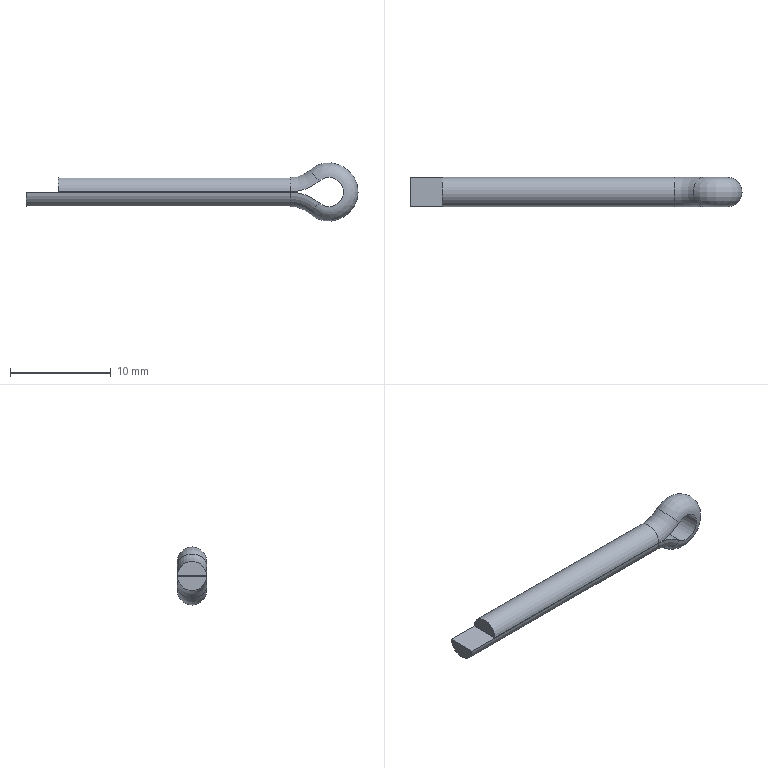Component | NX | COTTER_PIN_2_9X25_2 | 1 solid | 12 faces | box 33 x 2.9 x 5.72 mm | volume 211 mm3 | cylinder 5 | plane 4 | torus 2 | spline 1 | commonest cylinder face diameters 2.9 x2 8.69 x2 2.91 x1
STEP:
#1=VALUE_REPRESENTATION_ITEM('',COUNT_MEASURE(0.));
#2=(LENGTH_UNIT()NAMED_UNIT(*)SI_UNIT(.MILLI.,.METRE.));
#3=UNCERTAINTY_MEASURE_WITH_UNIT(LENGTH_MEASURE(0.0254),#2,'','');
#4=(NAMED_UNIT(*)PLANE_ANGLE_UNIT()SI_UNIT($,.RADIAN.));
#5=PLANE_ANGLE_MEASURE_WITH_UNIT(PLANE_ANGLE_MEASURE(0.01745),#4);
#6=DIMENSIONAL_EXPONENTS(0.,0.,0.,0.,0.,0.,0.);
#7=(CONVERSION_BASED_UNIT('',#5)NAMED_UNIT(#6)PLANE_ANGLE_UNIT());
#8=(NAMED_UNIT(*)SI_UNIT($,.STERADIAN.)SOLID_ANGLE_UNIT());
#9=(GEOMETRIC_REPRESENTATION_CONTEXT(3)GLOBAL_UNCERTAINTY_ASSIGNED_CONTEXT((#3))GLOBAL_UNIT_ASSIGNED_CONTEXT((#2,#7,#8))REPRESENTATION_CONTEXT('',''));
#10=REPRESENTATION('',(#1),#9);
#11=VALUE_REPRESENTATION_ITEM('',COUNT_MEASURE(0.));
#12=REPRESENTATION('',(#11),#9);
#13=CARTESIAN_POINT('',(0.,0.,0.));
#14=DIRECTION('',(0.,0.,1.));
#15=DIRECTION('',(1.,0.,0.));
#16=AXIS2_PLACEMENT_3D('',#13,#14,#15);
#17=SHAPE_REPRESENTATION('',(#16),#9);
#18=CARTESIAN_POINT('',(10.982,22.05,135.805));
#19=VERTEX_POINT('',#18);
#20=CARTESIAN_POINT('',(10.982,24.95,135.805));
#21=VERTEX_POINT('',#20);
#22=CARTESIAN_POINT('',(10.982,22.05,135.805));
#23=DIRECTION('',(0.,1.,0.));
#24=VECTOR('',#23,1.);
#25=LINE('',#22,#24);
#26=EDGE_CURVE('',#19,#21,#25,.T.);
#27=ORIENTED_EDGE('',*,*,#26,.T.);
#28=CARTESIAN_POINT('',(-15.3,24.95,135.805));
#29=VERTEX_POINT('',#28);
#30=CARTESIAN_POINT('',(10.982,24.95,135.805));
#31=DIRECTION('',(-1.,0.,0.));
#32=VECTOR('',#31,1.);
#33=LINE('',#30,#32);
#34=EDGE_CURVE('',#21,#29,#33,.T.);
#35=ORIENTED_EDGE('',*,*,#34,.T.);
#36=CARTESIAN_POINT('',(-15.3,22.05,135.805));
#37=VERTEX_POINT('',#36);
#38=CARTESIAN_POINT('',(-15.3,22.05,135.805));
#39=DIRECTION('',(0.,1.,0.));
#40=VECTOR('',#39,1.);
#41=LINE('',#38,#40);
#42=EDGE_CURVE('',#37,#29,#41,.T.);
#43=ORIENTED_EDGE('',*,*,#42,.F.);
#44=CARTESIAN_POINT('',(10.982,22.05,135.805));
#45=DIRECTION('',(-1.,0.,0.));
#46=VECTOR('',#45,1.);
#47=LINE('',#44,#46);
#48=EDGE_CURVE('',#19,#37,#47,.T.);
#49=ORIENTED_EDGE('',*,*,#48,.F.);
#50=EDGE_LOOP('',(#27,#35,#43,#49));
#51=FACE_OUTER_BOUND('',#50,.T.);
#52=CARTESIAN_POINT('',(10.982,22.05,135.805));
#53=DIRECTION('',(0.,0.,1.));
#54=DIRECTION('',(1.,0.,0.));
#55=AXIS2_PLACEMENT_3D('',#52,#53,#54);
#56=PLANE('',#55);
#57=ADVANCED_FACE('',(#51),#56,.T.);
#58=CARTESIAN_POINT('',(10.982,23.5,135.81));
#59=DIRECTION('',(-1.,0.,-0.));
#60=DIRECTION('',(0.,1.,0.));
#61=AXIS2_PLACEMENT_3D('',#58,#59,#60);
#62=CIRCLE('',#61,1.45);
#63=EDGE_CURVE('',#21,#19,#62,.T.);
#64=ORIENTED_EDGE('',*,*,#63,.T.);
#65=ORIENTED_EDGE('',*,*,#48,.T.);
#66=CARTESIAN_POINT('',(-15.3,23.5,135.81));
#67=DIRECTION('',(-1.,0.,-0.));
#68=DIRECTION('',(0.,1.,0.));
#69=AXIS2_PLACEMENT_3D('',#66,#67,#68);
#70=CIRCLE('',#69,1.45);
#71=EDGE_CURVE('',#29,#37,#70,.T.);
#72=ORIENTED_EDGE('',*,*,#71,.F.);
#73=ORIENTED_EDGE('',*,*,#34,.F.);
#74=EDGE_LOOP('',(#64,#65,#72,#73));
#75=FACE_OUTER_BOUND('',#74,.T.);
#76=CARTESIAN_POINT('',(10.982,23.5,135.81));
#77=DIRECTION('',(-1.,0.,0.));
#78=DIRECTION('',(0.,-1.,0.));
#79=AXIS2_PLACEMENT_3D('',#76,#77,#78);
#80=CYLINDRICAL_SURFACE('',#79,1.45);
#81=ADVANCED_FACE('',(#75),#80,.T.);
#82=CARTESIAN_POINT('',(13.856,22.05,134.719));
#83=VERTEX_POINT('',#82);
#84=CARTESIAN_POINT('',(13.856,24.95,134.719));
#85=VERTEX_POINT('',#84);
#86=CARTESIAN_POINT('',(13.856,22.05,134.719));
#87=DIRECTION('',(0.,1.,0.));
#88=VECTOR('',#87,1.);
#89=LINE('',#86,#88);
#90=EDGE_CURVE('',#83,#85,#89,.T.);
#91=ORIENTED_EDGE('',*,*,#90,.T.);
#92=CARTESIAN_POINT('',(10.982,24.95,131.46));
#93=DIRECTION('',(0.,-1.,0.));
#94=DIRECTION('',(1.,0.,0.));
#95=AXIS2_PLACEMENT_3D('',#92,#93,#94);
#96=CIRCLE('',#95,4.345);
#97=EDGE_CURVE('',#85,#21,#96,.T.);
#98=ORIENTED_EDGE('',*,*,#97,.T.);
#99=ORIENTED_EDGE('',*,*,#26,.F.);
#100=CARTESIAN_POINT('',(10.982,22.05,131.46));
#101=DIRECTION('',(0.,-1.,0.));
#102=DIRECTION('',(1.,0.,0.));
#103=AXIS2_PLACEMENT_3D('',#100,#101,#102);
#104=CIRCLE('',#103,4.345);
#105=EDGE_CURVE('',#83,#19,#104,.T.);
#106=ORIENTED_EDGE('',*,*,#105,.F.);
#107=EDGE_LOOP('',(#91,#98,#99,#106));
#108=FACE_OUTER_BOUND('',#107,.T.);
#109=CARTESIAN_POINT('',(10.982,23.5,131.46));
#110=DIRECTION('',(0.,-1.,0.));
#111=DIRECTION('',(1.,0.,0.));
#112=AXIS2_PLACEMENT_3D('',#109,#110,#111);
#113=CYLINDRICAL_SURFACE('',#112,4.345);
#114=ADVANCED_FACE('',(#108),#113,.T.);
#115=CARTESIAN_POINT('',(13.859,23.5,134.722));
#116=DIRECTION('',(-0.75,0.,0.6614));
#117=DIRECTION('',(0.,1.,0.));
#118=AXIS2_PLACEMENT_3D('',#115,#116,#117);
#119=CIRCLE('',#118,1.45);
#120=EDGE_CURVE('',#85,#83,#119,.T.);
#121=ORIENTED_EDGE('',*,*,#120,.T.);
#122=ORIENTED_EDGE('',*,*,#105,.T.);
#123=ORIENTED_EDGE('',*,*,#63,.F.);
#124=ORIENTED_EDGE('',*,*,#97,.F.);
#125=EDGE_LOOP('',(#121,#122,#123,#124));
#126=FACE_OUTER_BOUND('',#125,.T.);
#127=CARTESIAN_POINT('',(10.982,23.5,131.46));
#128=DIRECTION('',(0.,-1.,0.));
#129=DIRECTION('',(1.,0.,0.));
#130=AXIS2_PLACEMENT_3D('',#127,#128,#129);
#131=TOROIDAL_SURFACE('',#130,4.35,1.45);
#132=ADVANCED_FACE('',(#126),#131,.T.);
#133=CARTESIAN_POINT('',(13.856,22.05,136.901));
#134=VERTEX_POINT('',#133);
#135=CARTESIAN_POINT('',(13.856,24.95,136.901));
#136=VERTEX_POINT('',#135);
#137=CARTESIAN_POINT('',(13.856,22.05,136.901));
#138=DIRECTION('',(0.,1.,0.));
#139=VECTOR('',#138,1.);
#140=LINE('',#137,#139);
#141=EDGE_CURVE('',#134,#136,#140,.T.);
#142=ORIENTED_EDGE('',*,*,#141,.T.);
#143=CARTESIAN_POINT('',(14.818,24.95,135.81));
#144=DIRECTION('',(0.,1.,0.));
#145=DIRECTION('',(-1.,0.,0.));
#146=AXIS2_PLACEMENT_3D('',#143,#144,#145);
#147=CIRCLE('',#146,1.455);
#148=EDGE_CURVE('',#136,#85,#147,.T.);
#149=ORIENTED_EDGE('',*,*,#148,.T.);
#150=ORIENTED_EDGE('',*,*,#90,.F.);
#151=CARTESIAN_POINT('',(14.818,22.05,135.81));
#152=DIRECTION('',(0.,1.,0.));
#153=DIRECTION('',(-1.,0.,0.));
#154=AXIS2_PLACEMENT_3D('',#151,#152,#153);
#155=CIRCLE('',#154,1.455);
#156=EDGE_CURVE('',#134,#83,#155,.T.);
#157=ORIENTED_EDGE('',*,*,#156,.F.);
#158=EDGE_LOOP('',(#142,#149,#150,#157));
#159=FACE_OUTER_BOUND('',#158,.T.);
#160=CARTESIAN_POINT('',(14.818,23.5,135.81));
#161=DIRECTION('',(0.,1.,0.));
#162=DIRECTION('',(-1.,0.,0.));
#163=AXIS2_PLACEMENT_3D('',#160,#161,#162);
#164=CYLINDRICAL_SURFACE('',#163,1.455);
#165=ADVANCED_FACE('',(#159),#164,.F.);
#166=CARTESIAN_POINT('',(13.859,23.5,136.897));
#167=DIRECTION('',(0.75,0.,0.6614));
#168=DIRECTION('',(0.,1.,0.));
#169=AXIS2_PLACEMENT_3D('',#166,#167,#168);
#170=CIRCLE('',#169,1.45);
#171=EDGE_CURVE('',#136,#134,#170,.T.);
#172=ORIENTED_EDGE('',*,*,#171,.T.);
#173=ORIENTED_EDGE('',*,*,#156,.T.);
#174=ORIENTED_EDGE('',*,*,#120,.F.);
#175=ORIENTED_EDGE('',*,*,#148,.F.);
#176=EDGE_LOOP('',(#172,#173,#174,#175));
#177=FACE_OUTER_BOUND('',#176,.T.);
#178=CARTESIAN_POINT('',(13.856,24.95,136.901));
#179=CARTESIAN_POINT('',(14.947,24.95,137.863));
#180=CARTESIAN_POINT('',(16.273,24.95,137.265));
#181=CARTESIAN_POINT('',(16.273,24.95,135.81));
#182=CARTESIAN_POINT('',(16.273,24.95,134.355));
#183=CARTESIAN_POINT('',(14.947,24.95,133.756));
#184=CARTESIAN_POINT('',(13.856,24.95,134.719));
#185=CARTESIAN_POINT('',(11.951,24.94,139.061));
#186=CARTESIAN_POINT('',(15.202,24.94,141.929));
#187=CARTESIAN_POINT('',(19.153,24.94,140.145));
#188=CARTESIAN_POINT('',(19.153,24.94,135.81));
#189=CARTESIAN_POINT('',(19.153,24.94,131.475));
#190=CARTESIAN_POINT('',(15.202,24.94,129.691));
#191=CARTESIAN_POINT('',(11.951,24.94,132.559));
#192=CARTESIAN_POINT('',(11.951,22.06,139.061));
#193=CARTESIAN_POINT('',(15.202,22.06,141.929));
#194=CARTESIAN_POINT('',(19.153,22.06,140.145));
#195=CARTESIAN_POINT('',(19.153,22.06,135.81));
#196=CARTESIAN_POINT('',(19.153,22.06,131.475));
#197=CARTESIAN_POINT('',(15.202,22.06,129.691));
#198=CARTESIAN_POINT('',(11.951,22.06,132.559));
#199=CARTESIAN_POINT('',(13.856,22.05,136.901));
#200=CARTESIAN_POINT('',(14.947,22.05,137.863));
#201=CARTESIAN_POINT('',(16.273,22.05,137.265));
#202=CARTESIAN_POINT('',(16.273,22.05,135.81));
#203=CARTESIAN_POINT('',(16.273,22.05,134.355));
#204=CARTESIAN_POINT('',(14.947,22.05,133.756));
#205=CARTESIAN_POINT('',(13.856,22.05,134.719));
#206=(BOUNDED_SURFACE()B_SPLINE_SURFACE(3,3,((#178,#179,#180,#181,#182,#183,#184),(#185,#186,#187,#188,#189,#190,#191),(#192,#193,#194,#195,#196,#197,#198),(#199,#200,#201,#202,#203,#204,#205)),.UNSPECIFIED.,.F.,.F.,.F.)B_SPLINE_SURFACE_WITH_KNOTS((4,4),(4,3,4),(0.,1.),(0.,0.5,1.),.UNSPECIFIED.)GEOMETRIC_REPRESENTATION_ITEM()RATIONAL_B_SPLINE_SURFACE(((1.,0.6076,0.6076,1.,0.6076,0.6076,1.),(0.3356,0.2039,0.2039,0.3356,0.2039,0.2039,0.3356),(0.3356,0.2039,0.2039,0.3356,0.2039,0.2039,0.3356),(1.,0.6076,0.6076,1.,0.6076,0.6076,1.)))REPRESENTATION_ITEM('')SURFACE());
#207=ADVANCED_FACE('',(#177),#206,.T.);
#208=CARTESIAN_POINT('',(10.982,22.05,135.815));
#209=VERTEX_POINT('',#208);
#210=CARTESIAN_POINT('',(10.982,24.95,135.815));
#211=VERTEX_POINT('',#210);
#212=CARTESIAN_POINT('',(10.982,22.05,135.815));
#213=DIRECTION('',(0.,1.,0.));
#214=VECTOR('',#213,1.);
#215=LINE('',#212,#214);
#216=EDGE_CURVE('',#209,#211,#215,.T.);
#217=ORIENTED_EDGE('',*,*,#216,.T.);
#218=CARTESIAN_POINT('',(10.982,24.95,140.16));
#219=DIRECTION('',(0.,-1.,0.));
#220=DIRECTION('',(1.,0.,0.));
#221=AXIS2_PLACEMENT_3D('',#218,#219,#220);
#222=CIRCLE('',#221,4.345);
#223=EDGE_CURVE('',#211,#136,#222,.T.);
#224=ORIENTED_EDGE('',*,*,#223,.T.);
#225=ORIENTED_EDGE('',*,*,#141,.F.);
#226=CARTESIAN_POINT('',(10.982,22.05,140.16));
#227=DIRECTION('',(0.,-1.,0.));
#228=DIRECTION('',(1.,0.,0.));
#229=AXIS2_PLACEMENT_3D('',#226,#227,#228);
#230=CIRCLE('',#229,4.345);
#231=EDGE_CURVE('',#209,#134,#230,.T.);
#232=ORIENTED_EDGE('',*,*,#231,.F.);
#233=EDGE_LOOP('',(#217,#224,#225,#232));
#234=FACE_OUTER_BOUND('',#233,.T.);
#235=CARTESIAN_POINT('',(10.982,23.5,140.16));
#236=DIRECTION('',(0.,-1.,0.));
#237=DIRECTION('',(1.,0.,0.));
#238=AXIS2_PLACEMENT_3D('',#235,#236,#237);
#239=CYLINDRICAL_SURFACE('',#238,4.345);
#240=ADVANCED_FACE('',(#234),#239,.T.);
#241=CARTESIAN_POINT('',(10.982,23.5,135.81));
#242=DIRECTION('',(1.,0.,0.));
#243=DIRECTION('',(0.,1.,0.));
#244=AXIS2_PLACEMENT_3D('',#241,#242,#243);
#245=CIRCLE('',#244,1.45);
#246=EDGE_CURVE('',#211,#209,#245,.T.);
#247=ORIENTED_EDGE('',*,*,#246,.T.);
#248=ORIENTED_EDGE('',*,*,#231,.T.);
#249=ORIENTED_EDGE('',*,*,#171,.F.);
#250=ORIENTED_EDGE('',*,*,#223,.F.);
#251=EDGE_LOOP('',(#247,#248,#249,#250));
#252=FACE_OUTER_BOUND('',#251,.T.);
#253=CARTESIAN_POINT('',(10.982,23.5,140.16));
#254=DIRECTION('',(0.,-1.,0.));
#255=DIRECTION('',(1.,0.,0.));
#256=AXIS2_PLACEMENT_3D('',#253,#254,#255);
#257=TOROIDAL_SURFACE('',#256,4.35,1.45);
#258=ADVANCED_FACE('',(#252),#257,.T.);
#259=CARTESIAN_POINT('',(-12.1,24.95,135.815));
#260=VERTEX_POINT('',#259);
#261=CARTESIAN_POINT('',(-12.1,22.05,135.815));
#262=VERTEX_POINT('',#261);
#263=CARTESIAN_POINT('',(-12.1,23.5,135.81));
#264=DIRECTION('',(1.,0.,0.));
#265=DIRECTION('',(0.,1.,0.));
#266=AXIS2_PLACEMENT_3D('',#263,#264,#265);
#267=CIRCLE('',#266,1.45);
#268=EDGE_CURVE('',#260,#262,#267,.T.);
#269=ORIENTED_EDGE('',*,*,#268,.T.);
#270=CARTESIAN_POINT('',(10.982,22.05,135.815));
#271=DIRECTION('',(-1.,0.,0.));
#272=VECTOR('',#271,1.);
#273=LINE('',#270,#272);
#274=EDGE_CURVE('',#209,#262,#273,.T.);
#275=ORIENTED_EDGE('',*,*,#274,.F.);
#276=ORIENTED_EDGE('',*,*,#246,.F.);
#277=CARTESIAN_POINT('',(10.982,24.95,135.815));
#278=DIRECTION('',(-1.,0.,0.));
#279=VECTOR('',#278,1.);
#280=LINE('',#277,#279);
#281=EDGE_CURVE('',#211,#260,#280,.T.);
#282=ORIENTED_EDGE('',*,*,#281,.T.);
#283=EDGE_LOOP('',(#269,#275,#276,#282));
#284=FACE_OUTER_BOUND('',#283,.T.);
#285=CARTESIAN_POINT('',(10.982,23.5,135.81));
#286=DIRECTION('',(-1.,0.,0.));
#287=DIRECTION('',(0.,-1.,0.));
#288=AXIS2_PLACEMENT_3D('',#285,#286,#287);
#289=CYLINDRICAL_SURFACE('',#288,1.45);
#290=ADVANCED_FACE('',(#284),#289,.T.);
#291=CARTESIAN_POINT('',(-12.1,22.05,135.815));
#292=DIRECTION('',(0.,1.,0.));
#293=VECTOR('',#292,1.);
#294=LINE('',#291,#293);
#295=EDGE_CURVE('',#262,#260,#294,.T.);
#296=ORIENTED_EDGE('',*,*,#295,.T.);
#297=ORIENTED_EDGE('',*,*,#281,.F.);
#298=ORIENTED_EDGE('',*,*,#216,.F.);
#299=ORIENTED_EDGE('',*,*,#274,.T.);
#300=EDGE_LOOP('',(#296,#297,#298,#299));
#301=FACE_OUTER_BOUND('',#300,.T.);
#302=CARTESIAN_POINT('',(10.982,22.05,135.815));
#303=DIRECTION('',(0.,0.,1.));
#304=DIRECTION('',(1.,0.,0.));
#305=AXIS2_PLACEMENT_3D('',#302,#303,#304);
#306=PLANE('',#305);
#307=ADVANCED_FACE('',(#301),#306,.F.);
#308=ORIENTED_EDGE('',*,*,#71,.T.);
#309=ORIENTED_EDGE('',*,*,#42,.T.);
#310=EDGE_LOOP('',(#308,#309));
#311=FACE_OUTER_BOUND('',#310,.T.);
#312=CARTESIAN_POINT('',(-15.3,23.5,135.81));
#313=DIRECTION('',(-1.,0.,-0.));
#314=DIRECTION('',(0.,1.,0.));
#315=AXIS2_PLACEMENT_3D('',#312,#313,#314);
#316=PLANE('',#315);
#317=ADVANCED_FACE('',(#311),#316,.T.);
#318=ORIENTED_EDGE('',*,*,#268,.F.);
#319=ORIENTED_EDGE('',*,*,#295,.F.);
#320=EDGE_LOOP('',(#318,#319));
#321=FACE_OUTER_BOUND('',#320,.T.);
#322=CARTESIAN_POINT('',(-12.1,23.5,135.81));
#323=DIRECTION('',(1.,0.,0.));
#324=DIRECTION('',(0.,1.,0.));
#325=AXIS2_PLACEMENT_3D('',#322,#323,#324);
#326=PLANE('',#325);
#327=ADVANCED_FACE('',(#321),#326,.F.);
#328=CLOSED_SHELL('',(#57,#81,#114,#132,#165,#207,#240,#258,#290,#307,#317,#327));
#329=MANIFOLD_SOLID_BREP('',#328);
#330=ADVANCED_BREP_SHAPE_REPRESENTATION('',(#329),#9);
#331=SHAPE_REPRESENTATION_RELATIONSHIP('','',#17,#330);
#332=PRESENTATION_LAYER_ASSIGNMENT('','',(#329));
#333=COLOUR_RGB('',0.6,0.6,0.6);
#334=FILL_AREA_STYLE_COLOUR('',#333);
#335=FILL_AREA_STYLE('',(#334));
#336=SURFACE_STYLE_FILL_AREA(#335);
#337=SURFACE_SIDE_STYLE('',(#336));
#338=SURFACE_STYLE_USAGE(.BOTH.,#337);
#339=PRESENTATION_STYLE_ASSIGNMENT((#338));
#340=STYLED_ITEM('',(#339),#329);
#341=MECHANICAL_DESIGN_GEOMETRIC_PRESENTATION_REPRESENTATION('',(#340),#9);